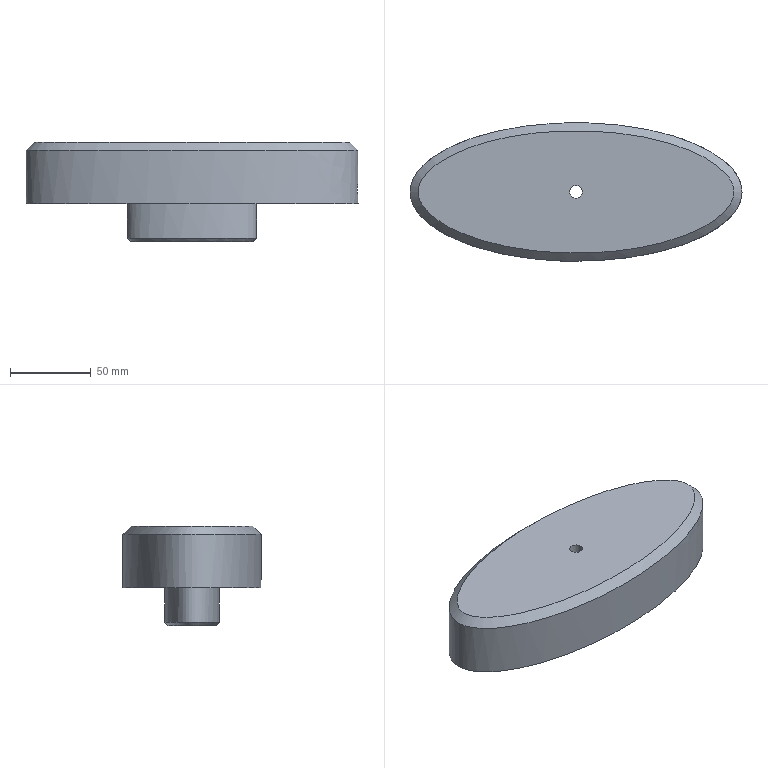Component | NX | LOCATING_BLOCK | 1 solid | 12 faces | volume 562076 mm3 | cylinder 3 | spline 3 | plane 3 | cone 2 | other 1 | commonest cylinder face diameters 8 x2 19.623 x1